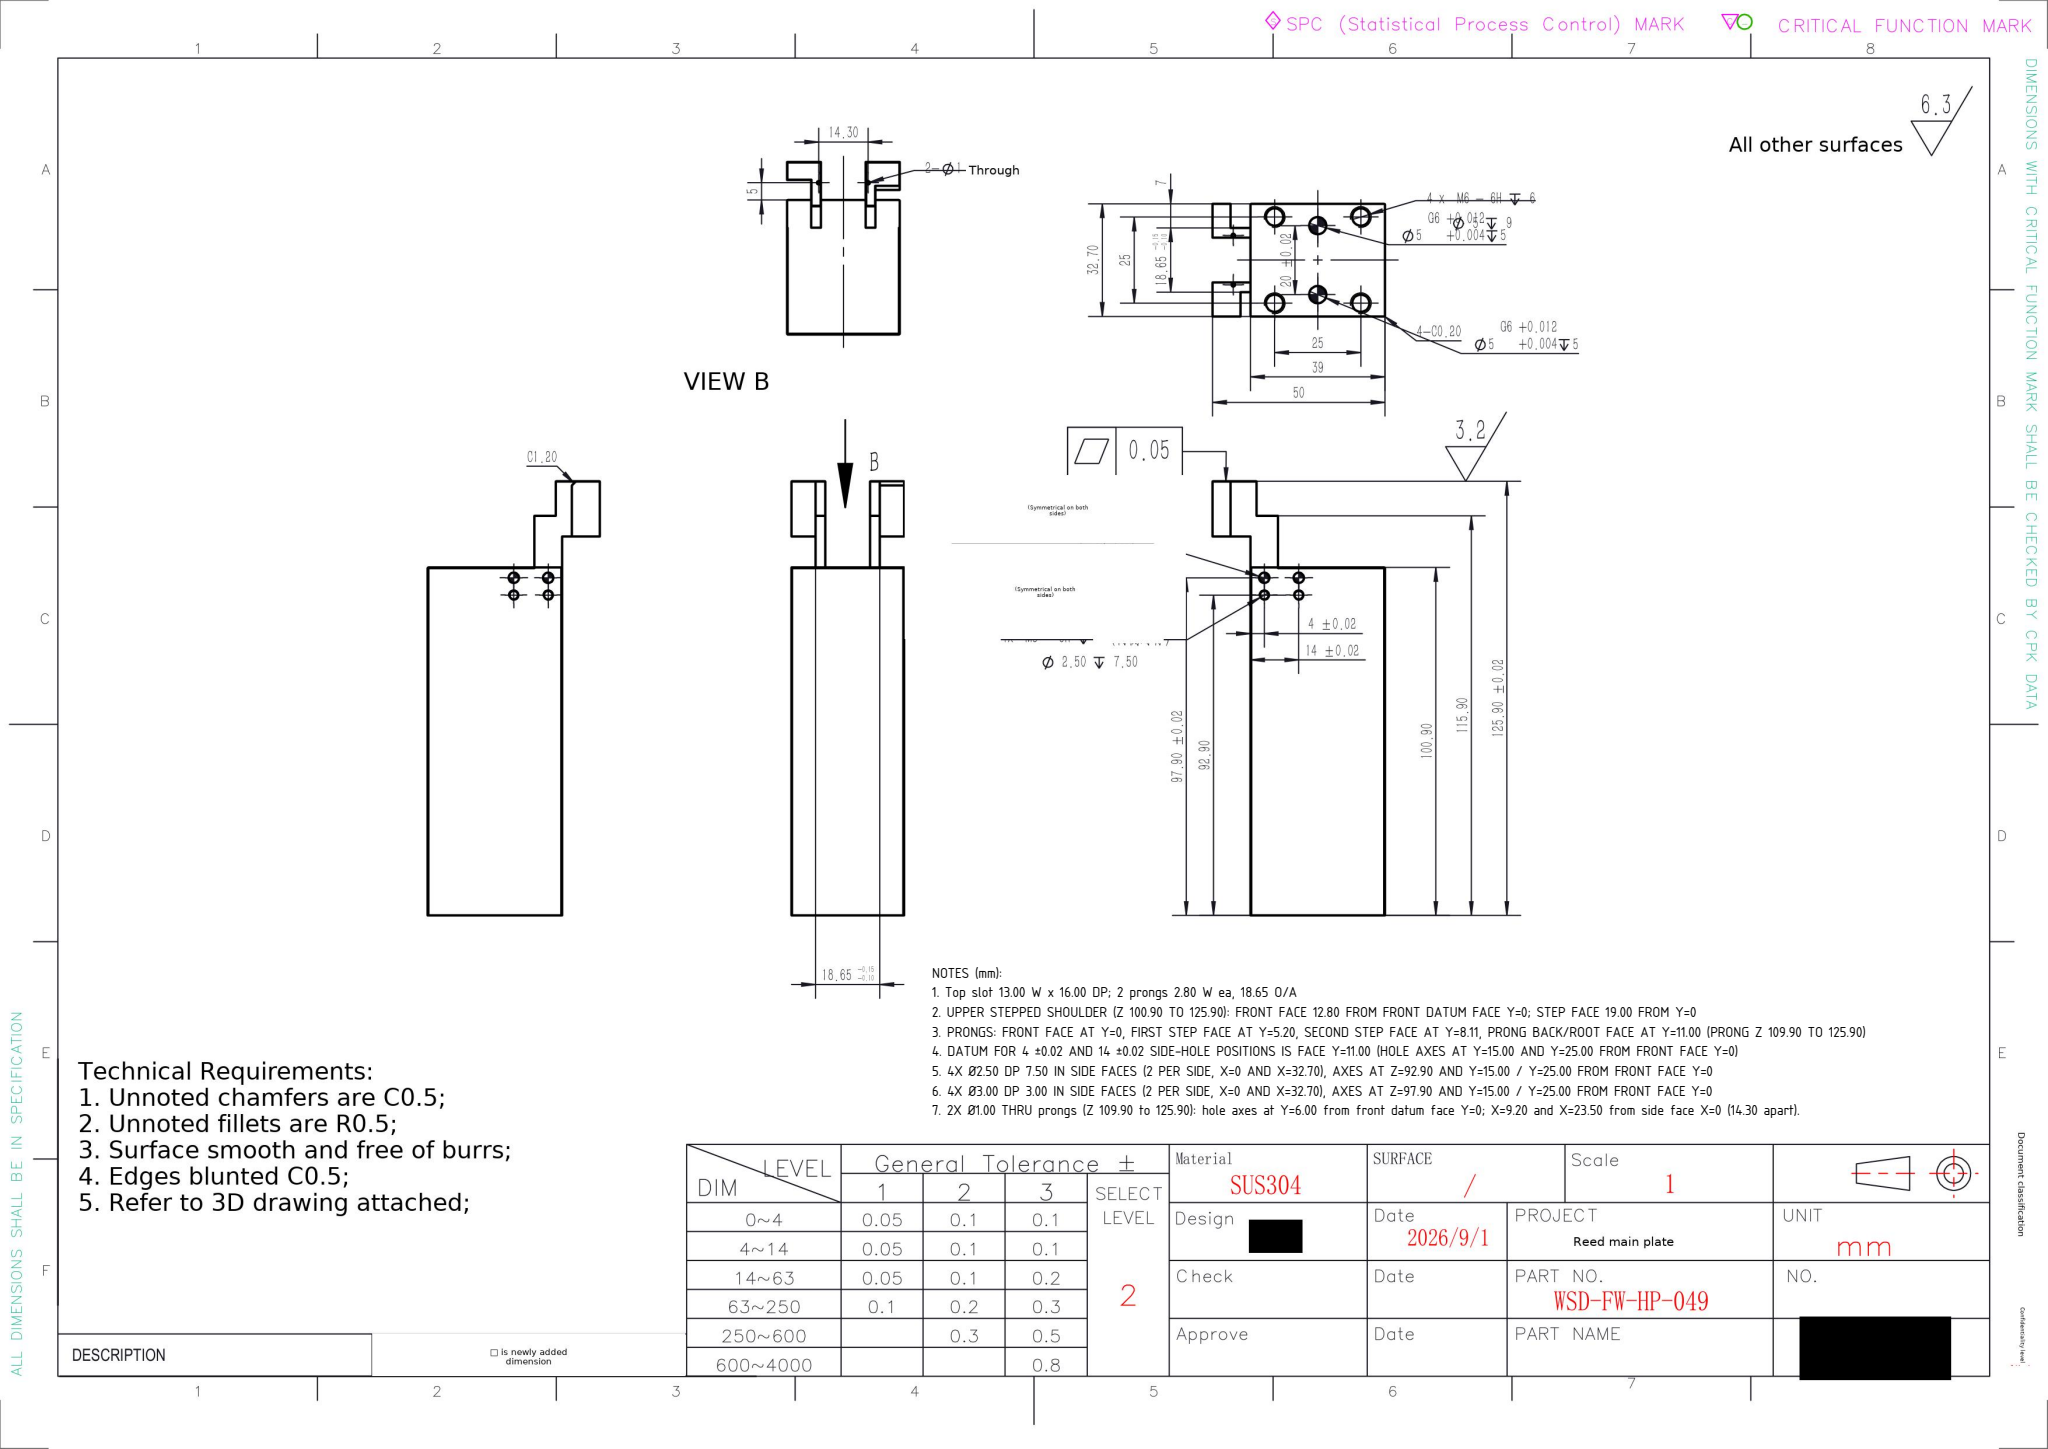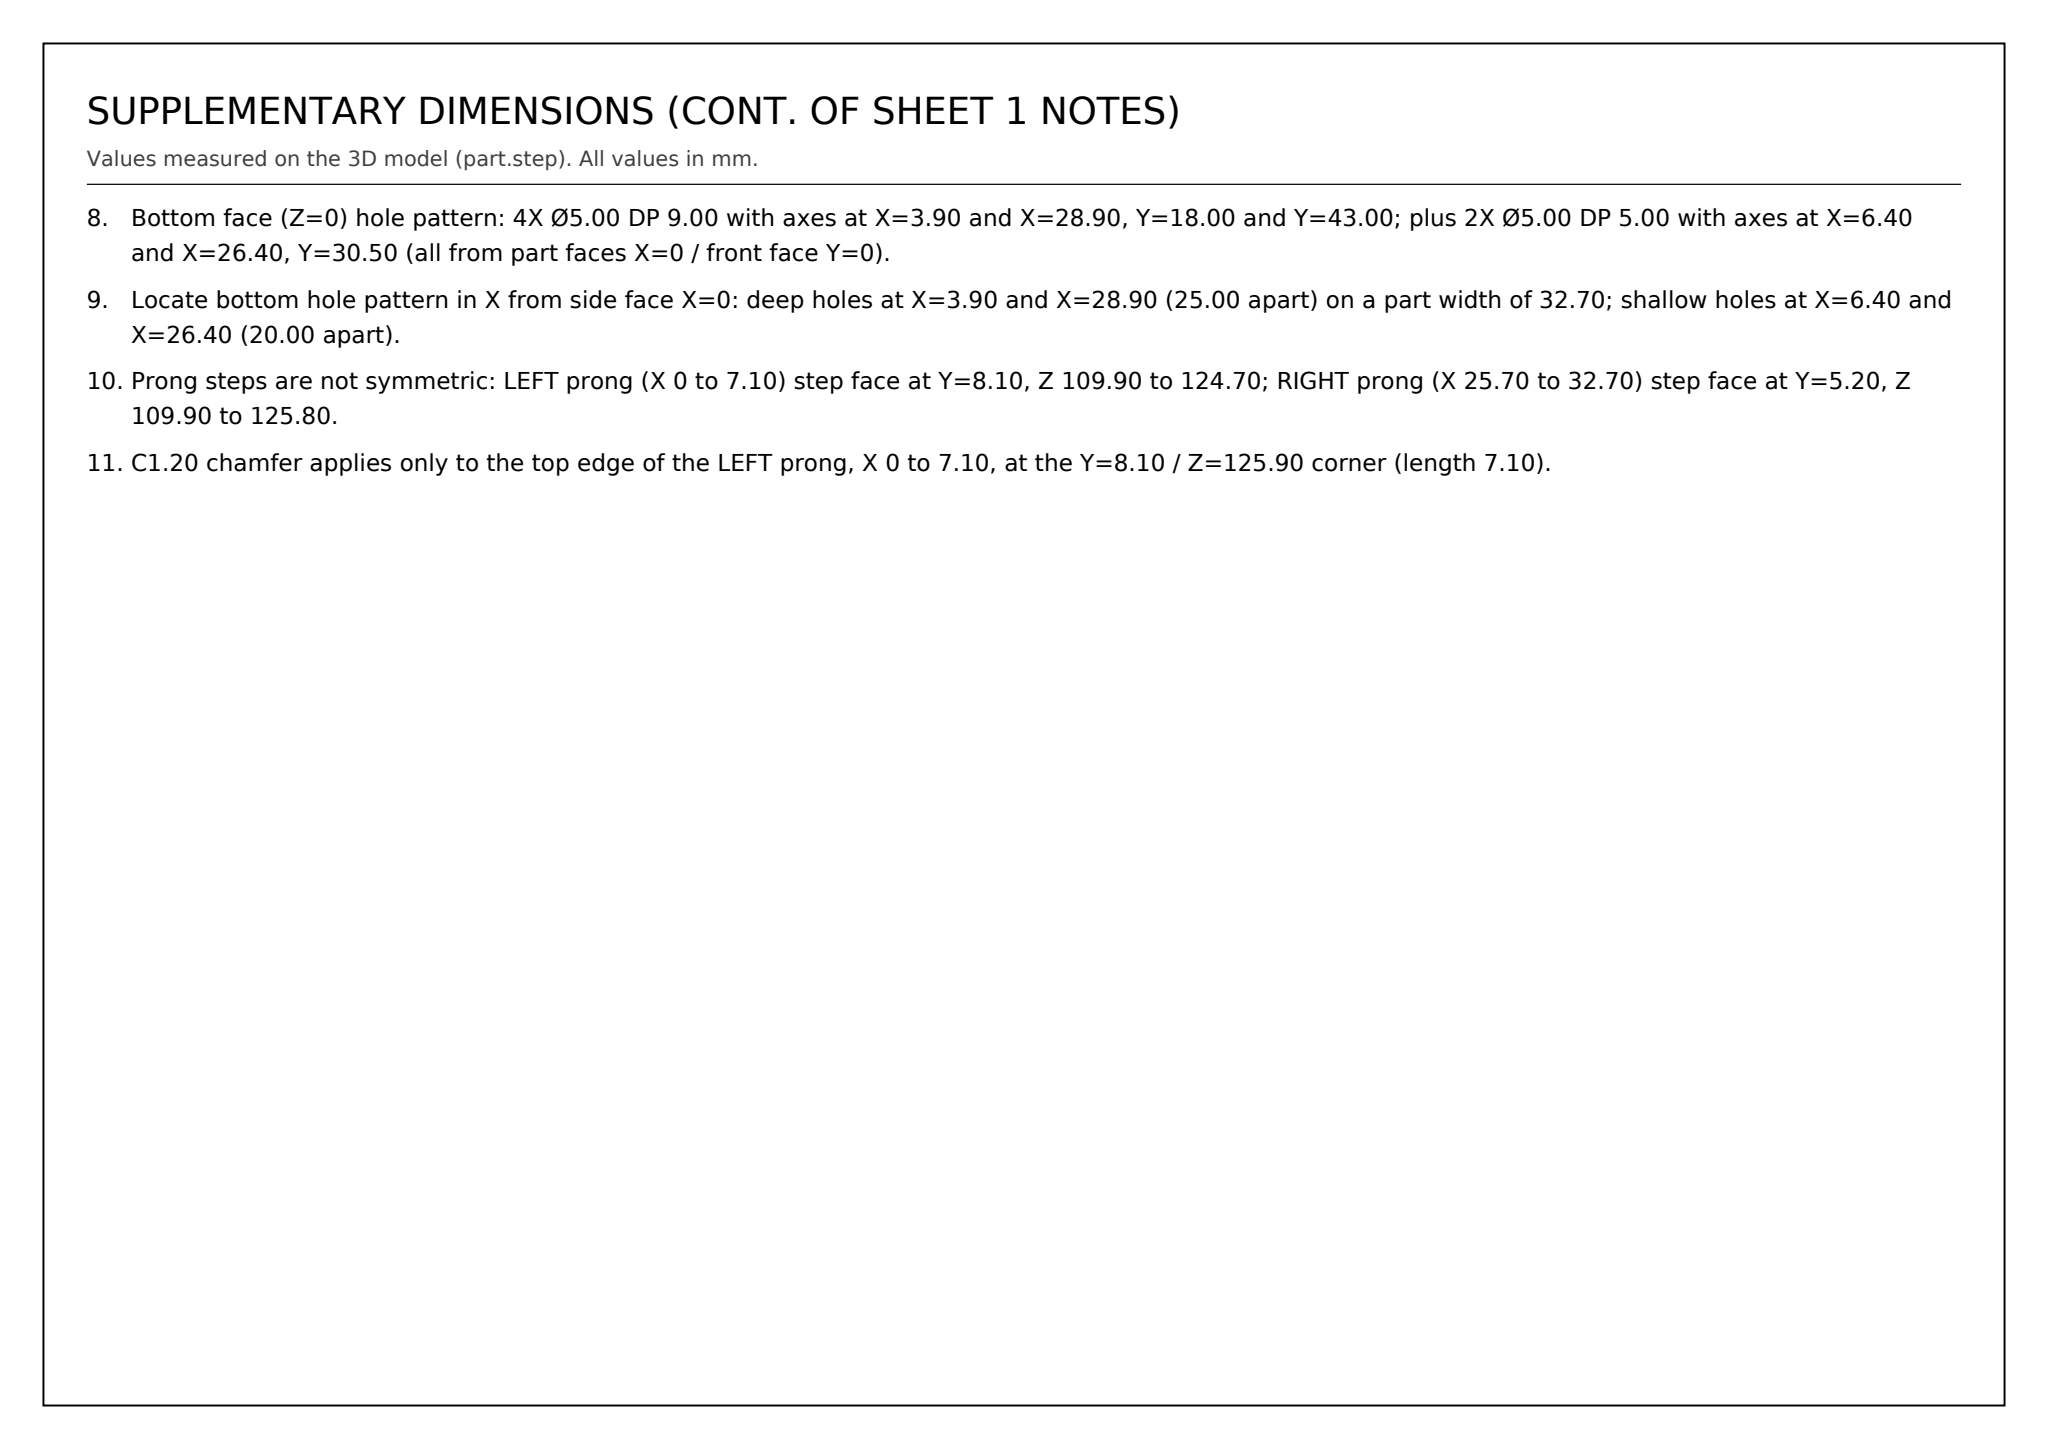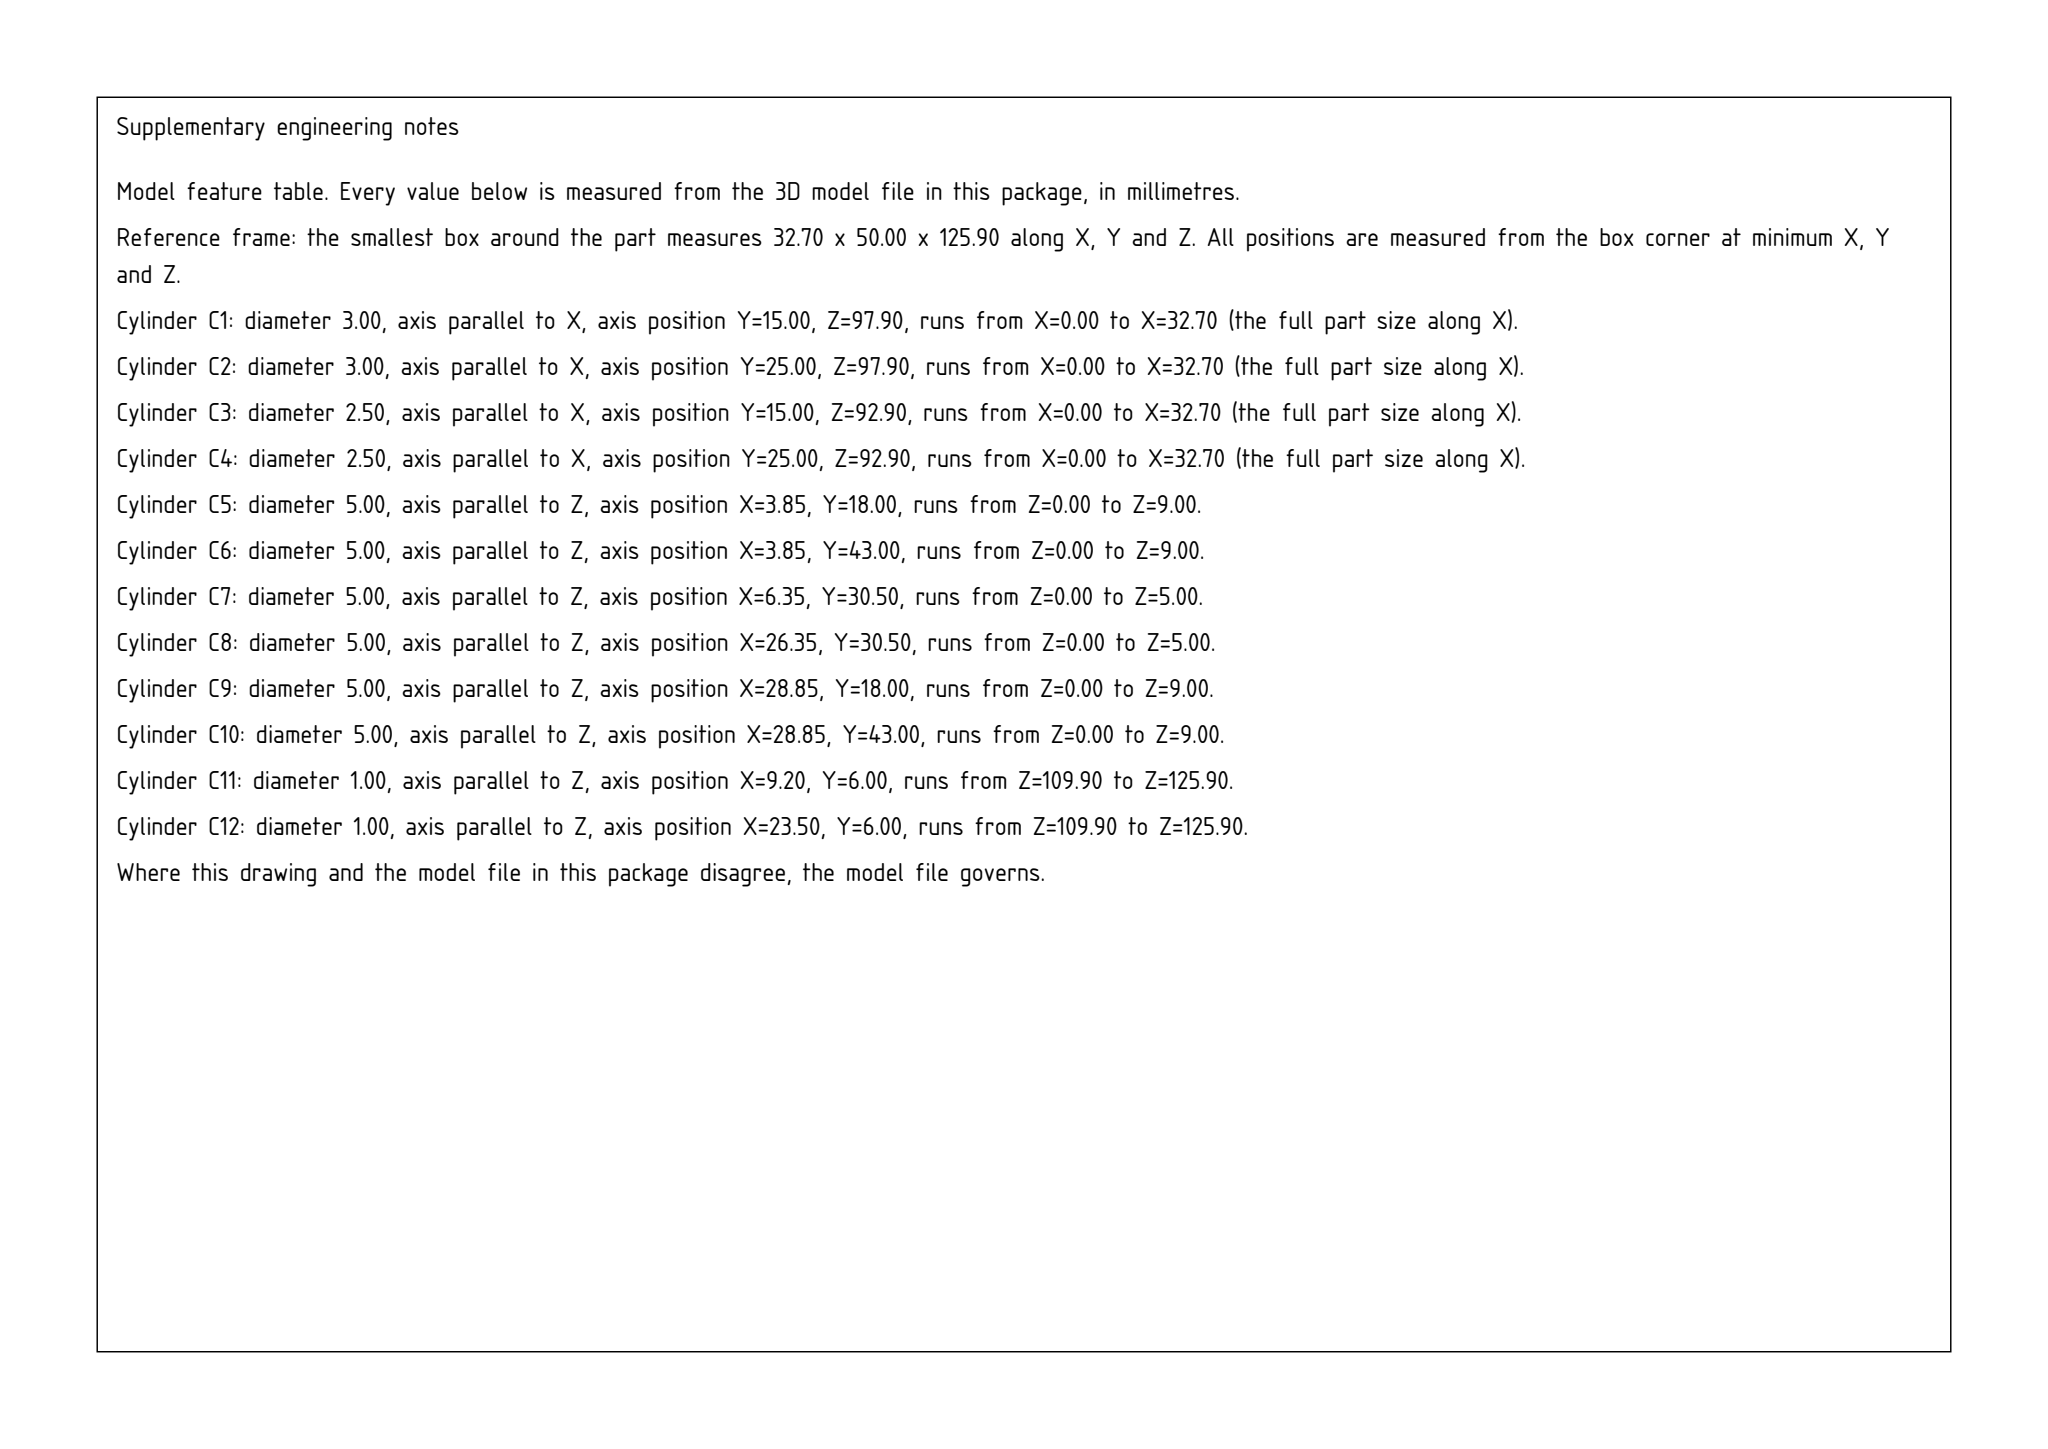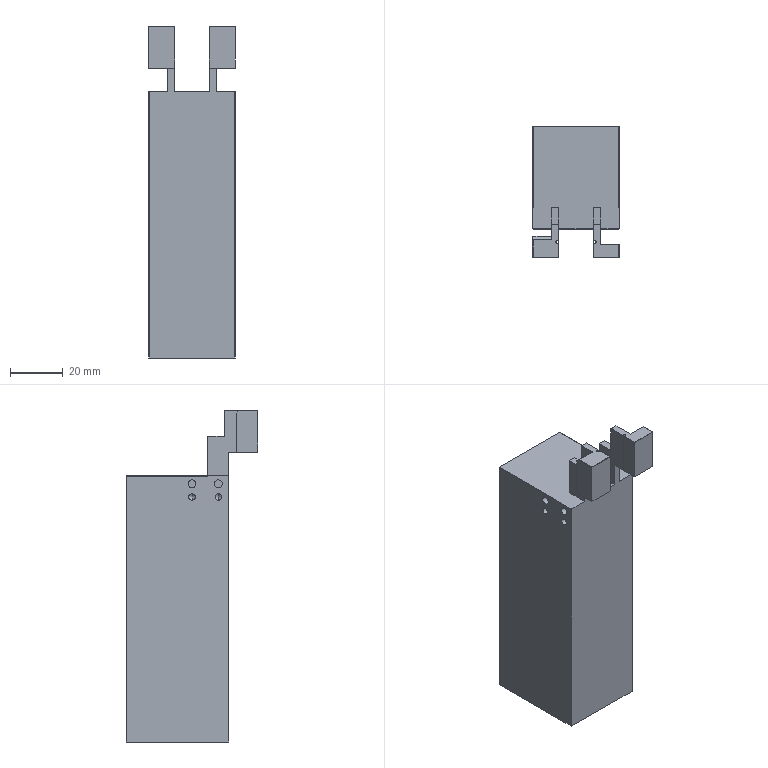Part | SolidWorks | mm | 1 solid | 103 faces | box 32.7 x 50 x 125.9 mm | volume 130729 mm3 | plane 55 | cylinder 32 | cone 16 | commonest cylinder face diameters 5 x12 2.5 x8 3 x8 1 x4
Drawing notes:
Top slot 13.00 W x 16.00 DP; 2 prongs 2.80 W ea, 18.65 O/A | from the solid: x planes 7.05/9.85/22.85/25.7: prong W 2.80 ea, gap 22.85-9.85=13.00, O/A 25.7-7.05=18.65; z 109.9-125.9=16.00 DP
UPPER STEPPED SHOULDER (Z 100.90 TO 125.90): FRONT FACE 12.80 FROM FRONT DATUM FACE Y=0; STEP FACE 19.00 FROM Y=0 | from the solid: axis_planes y=12.8 (2) and y=19.0 (4) with z planes 100.9 / 115.9 / 125.9
PRONGS: FRONT FACE AT Y=0, FIRST STEP FACE AT Y=5.20, SECOND STEP FACE AT Y=8.11, PRONG BACK/ROOT FACE AT Y=11.00 (PRONG Z 109.90 TO 125.90) | from the solid: axis_planes y=0, 5.2, 8.11, 11.0; z planes 109.9 and 125.9; prong x planes 7.05/9.85/22.85/25.70
DATUM FOR 4 ±0.02 AND 14 ±0.02 SIDE-HOLE POSITIONS IS FACE Y=11.00 (HOLE AXES AT Y=15.00 AND Y=25.00 FROM FRONT FACE Y=0) | from the solid: axis_plane y=11.0; Ø2.5 and Ø3.0 x-axis cylinders at y=15.0 and y=25.0
4X Ø2.50 DP 7.50 IN SIDE FACES (2 PER SIDE, X=0 AND X=32.70), AXES AT Z=92.90 AND Y=15.00 / Y=25.00 FROM FRONT FACE Y=0 | from the solid: cylinders [2.5,x,(y=15,z=92.9),len 7.5] and [2.5,x,(y=25,z=92.9),len 7.5]
4X Ø3.00 DP 3.00 IN SIDE FACES (2 PER SIDE, X=0 AND X=32.70), AXES AT Z=97.90 AND Y=15.00 / Y=25.00 FROM FRONT FACE Y=0 | from the solid: cylinders [3.0,x,(y=15,z=97.9),len 3.0] and [3.0,x,(y=25,z=97.9),len 3.0]
2X Ø1.00 THRU prongs (Z 109.90 to 125.90): hole axes at Y=6.00 from front datum face Y=0; X=9.20 and X=23.50 from side face X=0 (14.30 apart). | from the solid: cylinders: hole/bore Ø1.0 axis z at (x=9.2,y=6.0) and (x=23.5,y=6.0), from z=109.9 to 125.9
Bottom face (Z=0) hole pattern: 4X Ø5.00 DP 9.00 with axes at X=3.90 and X=28.90, Y=18.00 and Y=43.00; plus 2X Ø5.00 DP 5.00 with axes at X=6.40 and X=26.40, Y=30.50 (all from part faces X=0 / front face Y=0). | from the solid: cylinders: Ø5 z-axis at (3.9,18.0),(3.9,43.0),(28.9,18.0),(28.9,43.0) from z=0 to 9.0; Ø5 z-axis at (6.4,30.5),(26.4,30.5) from z=0 to 5.0
Locate bottom hole pattern in X from side face X=0: deep holes at X=3.90 and X=28.90 (25.00 apart) on a part width of 32.70; shallow holes at X=6.40 and X=26.40 (20.00 apart). | from the solid: bbox_xyz x=32.7; Ø5 hole axis x values 3.9/28.9 (↧9) and 6.4/26.4 (↧5)
Prong steps are not symmetric: LEFT prong (X 0 to 7.10) step face at Y=8.10, Z 109.90 to 124.70; RIGHT prong (X 25.70 to 32.70) step face at Y=5.20, Z 109.90 to 125.80. | from the solid: axis_planes: y=8.1 extent x[0.0,7.1] z[109.9,124.7]; y=5.2 extent x[25.7,32.7] z[109.9,125.8]
C1.20 chamfer applies only to the top edge of the LEFT prong, X 0 to 7.10, at the Y=8.10 / Z=125.90 corner (length 7.10). | from the solid: inclined_planes: angle [90,45,45], bbox_from [0.0,6.9,124.7], size [7.2,1.2,1.2]
build123d program:
from build123d import *

# Parameters (mm, degrees)
SKETCH1_W             = 32.7
SKETCH1_H             = 50
BOSS_EXTRUDE1_DEPTH   = 125.9
SKETCH10_W            = 13
SKETCH10_H            = 25
CUT_EXTRUDE5_DEPTH    = 137.448
SKETCH11_W            = 109.9
SKETCH11_H            = 11
CUT_EXTRUDE6_DEPTH    = 133.458
SKETCH15_W            = 25
SKETCH15_H            = 31
CUT_EXTRUDE8_DEPTH    = 133.458
M3_TAPPED_HOLE3_D     = 2.5
M3_TAPPED_HOLE3_DEPTH = 7.5
M3_TAPPED_HOLE3_TIP   = 0.7511
SKETCH18_R            = 1.5
CUT_EXTRUDE9_DEPTH    = 3
CUT_EXTRUDE10_START   = -3
SKETCH19_R            = 1.5
CUT_EXTRUDE10_DEPTH   = 3
M3_TAPPED_HOLE4_D     = 2.5
M3_TAPPED_HOLE4_DEPTH = 7.5
M3_TAPPED_HOLE4_TIP   = 0.7511
CHAMFER1_SIZE         = 0.2
SKETCH23_R            = 2.5
CUT_EXTRUDE12_DEPTH   = 5
M6_TAPPED_HOLE1_D     = 5
M6_TAPPED_HOLE1_DEPTH = 9
M6_TAPPED_HOLE1_TIP   = 1.502
CUT_EXTRUDE13_REACH   = 131.395
SKETCH26_W            = 7
SKETCH26_H            = 13.8
SKETCH26_W_2          = 7.05
SKETCH26_H_2          = 10.89
SKETCH31_W            = 51.841
SKETCH31_H            = 14.292
CUT_EXTRUDE16_DEPTH   = 10
CHAMFER2_SIZE         = 0.1
CHAMFER3_SIZE         = 1.2
SKETCH32_R            = 0.5
CUT_EXTRUDE17_DEPTH   = 130.395


with BuildPart() as part:
    # Sketch1 → Boss-Extrude1 (new body)
    with BuildSketch(Plane.XY):
        Rectangle(SKETCH1_W, SKETCH1_H)
    extrude(amount=BOSS_EXTRUDE1_DEPTH)

    # Sketch10 → Cut-Extrude5 (cut, through all)
    with BuildSketch(Plane.XZ.offset(25)):
        with Locations((0, 113.4)):
            Rectangle(SKETCH10_W, SKETCH10_H)
    extrude(amount=-CUT_EXTRUDE5_DEPTH, mode=Mode.SUBTRACT)

    # Sketch11 → Cut-Extrude6 (cut, through all)
    with BuildSketch(Plane(origin=(16.35, 0, 0), x_dir=(0, 0, -1), z_dir=(1, 0, 0))):
        with Locations((-54.95, -19.5)):
            Rectangle(SKETCH11_W, SKETCH11_H)
    extrude(amount=-CUT_EXTRUDE6_DEPTH, mode=Mode.SUBTRACT)

    # Sketch15 → Cut-Extrude8 (cut, through all)
    with BuildSketch(Plane(origin=(16.35, 0, 0), x_dir=(0, 0, -1), z_dir=(1, 0, 0))):
        with Locations((-113.4, 9.5)):
            Rectangle(SKETCH15_W, SKETCH15_H)
    extrude(amount=-CUT_EXTRUDE8_DEPTH, mode=Mode.SUBTRACT)

    # M3 Tapped Hole3
    with Locations(Plane(origin=(16.35, 0, 0), x_dir=(0, 0, -1), z_dir=(1, 0, 0))):
        with Locations((-92.9, 0), (-92.9, -10)):
            Hole(M3_TAPPED_HOLE3_D / 2, depth=M3_TAPPED_HOLE3_DEPTH)
            with Locations((0, 0, -(M3_TAPPED_HOLE3_DEPTH + M3_TAPPED_HOLE3_TIP / 2))):  # 118° drill point
                Cone(0, M3_TAPPED_HOLE3_D / 2, M3_TAPPED_HOLE3_TIP, mode=Mode.SUBTRACT)

    # Sketch18 → Cut-Extrude9 (cut)
    with BuildSketch(Plane(origin=(16.35, 0, 0), x_dir=(0, 0, -1), z_dir=(1, 0, 0))):
        with Locations(Location((-97.9, 0, 0), (0, 0, 90))):
            Circle(SKETCH18_R)
        with Locations(Location((-97.9, -10, 0), (0, 0, 90))):
            Circle(SKETCH18_R)
    extrude(amount=-CUT_EXTRUDE9_DEPTH, mode=Mode.SUBTRACT)

    # Sketch19 → Cut-Extrude10 (cut)
    with BuildSketch(Plane.ZY.offset(16.35).offset(CUT_EXTRUDE10_START)):
        with Locations(Location((97.9, 0, 0), (0, 0, 90))):
            Circle(SKETCH19_R)
        with Locations(Location((97.9, -10, 0), (0, 0, 90))):
            Circle(SKETCH19_R)
    extrude(amount=CUT_EXTRUDE10_DEPTH, mode=Mode.SUBTRACT)

    # M3 Tapped Hole4
    with Locations(Plane.ZY.offset(16.35)):
        with Locations((92.9, 0), (92.9, -10)):
            Hole(M3_TAPPED_HOLE4_D / 2, depth=M3_TAPPED_HOLE4_DEPTH)
            with Locations((0, 0, -(M3_TAPPED_HOLE4_DEPTH + M3_TAPPED_HOLE4_TIP / 2))):  # 118° drill point
                Cone(0, M3_TAPPED_HOLE4_D / 2, M3_TAPPED_HOLE4_TIP, mode=Mode.SUBTRACT)

    # Chamfer1
    chamfer1_edges = [part.edges().sort_by_distance(p)[0] for p in [
        (0, 25, 100.9),
        (-16.35, -14, 54.95),
        (16.35, -14, 54.95),
        (-16.35, 25, 50.45),
        (16.35, 25, 50.45),
        (16.35, 9.5, 100.9),
        (-11.425, -6, 125.9),
        (11.425, -6, 125.9),
        (-16.35, 9.5, 100.9),
    ]]
    chamfer(chamfer1_edges, length=CHAMFER1_SIZE)

    # Sketch23 → Cut-Extrude12 (cut)
    with BuildSketch(Plane(origin=(0, 0, 0), x_dir=(-1, 0, 0), z_dir=(0, 0, -1))):
        with Locations((-10, 5.5)):
            Circle(SKETCH23_R)
        with Locations(Location((10, 5.5, 0), (0, 0, 180))):
            Circle(SKETCH23_R)
    extrude(amount=-CUT_EXTRUDE12_DEPTH, mode=Mode.SUBTRACT)

    # M6 Tapped Hole1
    with Locations(Plane(origin=(0, 0, 0), x_dir=(-1, 0, 0), z_dir=(0, 0, -1))):
        with Locations((-12.5, 18), (12.5, 18), (12.5, -7), (-12.5, -7)):
            Hole(M6_TAPPED_HOLE1_D / 2, depth=M6_TAPPED_HOLE1_DEPTH)
            with Locations((0, 0, -(M6_TAPPED_HOLE1_DEPTH + M6_TAPPED_HOLE1_TIP / 2))):  # 118° drill point
                Cone(0, M6_TAPPED_HOLE1_D / 2, M6_TAPPED_HOLE1_TIP, mode=Mode.SUBTRACT)

    # Cut-Extrude13: up to this face of the body (flat: up to its plane)
    cut_extrude13_end = Plane(part.part.faces().sort_by_distance((0, 7.564, 100.9))[0])
    # Sketch26 → Cut-Extrude13 (cut, up to the picked face)
    with BuildSketch(Plane.XY.offset(125.9), mode=Mode.PRIVATE) as cut_extrude13_sk1:
        with Locations((12.85, -12.9)):
            Rectangle(SKETCH26_W, SKETCH26_H)
    cut_extrude13_tool1 = split(extrude(cut_extrude13_sk1.sketch, amount=-CUT_EXTRUDE13_REACH, mode=Mode.PRIVATE), bisect_by=cut_extrude13_end, keep=Keep.BOTH, mode=Mode.PRIVATE)
    # Sketch26 → Cut-Extrude13 (cut, up to the picked face)
    with BuildSketch(Plane.XY.offset(125.9), mode=Mode.PRIVATE) as cut_extrude13_sk2:
        with Locations((-12.825, -11.445)):
            Rectangle(SKETCH26_W_2, SKETCH26_H_2)
    cut_extrude13_tool2 = split(extrude(cut_extrude13_sk2.sketch, amount=-CUT_EXTRUDE13_REACH, mode=Mode.PRIVATE), bisect_by=cut_extrude13_end, keep=Keep.BOTH, mode=Mode.PRIVATE)
    add(cut_extrude13_tool1.solids().sort_by(Axis((12.85, -12.9, 125.9), (0, 0, -1)))[0], mode=Mode.SUBTRACT)
    add(cut_extrude13_tool2.solids().sort_by(Axis((-12.825, -11.445, 125.9), (0, 0, -1)))[0], mode=Mode.SUBTRACT)

    # Sketch31 → Cut-Extrude16 (cut)
    with BuildSketch(Plane.XY.offset(125.9)):
        with Locations((-0.01535, -5.054)):
            Rectangle(SKETCH31_W, SKETCH31_H)
    extrude(amount=-CUT_EXTRUDE16_DEPTH, mode=Mode.SUBTRACT)

    # Chamfer2
    chamfer2_edges = [part.edges().sort_by_distance(p)[0] for p in [
        (-11.425, -25, 125.9),
        (11.425, -25, 125.9),
        (12.85, -19.8, 125.9),
        (-16.35, -20.945, 125.9),
        (-9.3, -14.545, 125.9),
        (9.35, -16, 125.9),
        (6.5, -18.6, 125.9),
        (-6.5, -18.6, 125.9),
        (7.925, -12.2, 125.9),
        (-7.9, -12.2, 125.9),
        (16.35, -22.4, 125.9),
    ]]
    chamfer(chamfer2_edges, length=CHAMFER2_SIZE)

    # Chamfer3
    chamfer3_edges = [part.edges().sort_by_distance(p)[0] for p in [
        (-12.725, -16.89, 125.9),
    ]]
    chamfer(chamfer3_edges, length=CHAMFER3_SIZE)

    # Sketch32 → Cut-Extrude17 (cut, through all)
    with BuildSketch(Plane.XY.offset(125.9)):
        with Locations((7.15, -19)):
            Circle(SKETCH32_R)
        with Locations((-7.15, -19)):
            Circle(SKETCH32_R)
    extrude(amount=-CUT_EXTRUDE17_DEPTH, mode=Mode.SUBTRACT)


solid = part.part